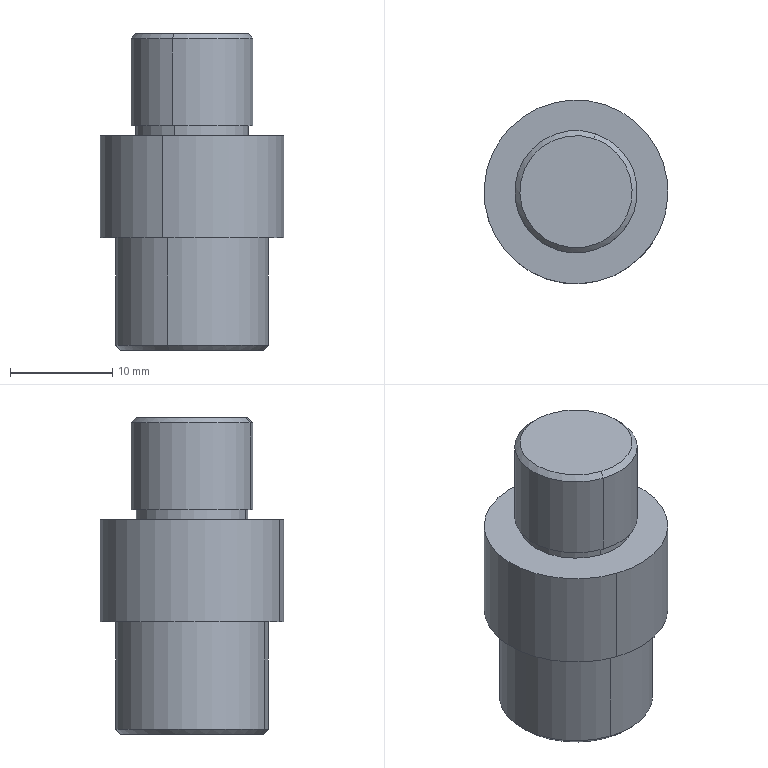Component | SolidWorks | 01-02WheelAxis-2 | 1 solid | 21 faces | box 18 x 18 x 31 mm | volume 5093 mm3 | cylinder 10 | cone 6 | plane 5 | commonest cylinder face diameters 6 x2 12 x2 11 x2 18 x2 15 x2 | material 45
build123d program:
from build123d import *

# Parameters (mm, degrees)
CHAMFER1_SIZE         = 0.5
M6_TAPPED_HOLE1_D     = 6
M6_TAPPED_HOLE1_DEPTH = 17
M6_TAPPED_HOLE1_TIP   = 1.803


with BuildPart() as part:
    # Sketch1 → Revolve1 (revolve)
    with BuildSketch(Plane.XY, mode=Mode.PRIVATE) as revolve1_sk:
        Polygon((0, 6), (0, 0), (31, 0), (31, 7.5), (20, 7.5), (20, 9), (10, 9), (10, 6), (10, 5.5), (9, 5.5), (9, 6), align=None)
    revolve(revolve1_sk.sketch.rotate(Axis((31, 0, 0), (-1, 0, 0)), 90), axis=Axis((31, 0, 0), (-1, 0, 0)))

    # Chamfer1
    chamfer1_edges = [part.edges().sort_by_distance(p)[0] for p in [
        (31, 0, 7.5),
        (0, 0, 6),
    ]]
    chamfer(chamfer1_edges, length=CHAMFER1_SIZE)

    # M6 Tapped Hole1
    with Locations(Plane(origin=(31, 0, 0), x_dir=(0, 0, -1), z_dir=(1, 0, 0))):
        with Locations((0, 0)):
            Hole(M6_TAPPED_HOLE1_D / 2, depth=M6_TAPPED_HOLE1_DEPTH)
            with Locations((0, 0, -(M6_TAPPED_HOLE1_DEPTH + M6_TAPPED_HOLE1_TIP / 2))):  # 118° drill point
                Cone(0, M6_TAPPED_HOLE1_D / 2, M6_TAPPED_HOLE1_TIP, mode=Mode.SUBTRACT)


solid = part.part

# Placed as in the assembly
solid = solid.moved(Location((300, -53.25, -443), (0, 90, 0)))
STEP:
#1=COLOUR_RGB('',0.7922,0.8196,0.9333);
#2=FILL_AREA_STYLE_COLOUR('',#1);
#3=FILL_AREA_STYLE('',(#2));
#4=SURFACE_STYLE_FILL_AREA(#3);
#5=SURFACE_SIDE_STYLE('',(#4));
#6=SURFACE_STYLE_USAGE(.BOTH.,#5);
#7=PRESENTATION_STYLE_ASSIGNMENT((#6));
#8=CARTESIAN_POINT('',(11.773,-2.208,-17.992));
#9=VERTEX_POINT('',#8);
#10=CARTESIAN_POINT('',(11.849,-1.985,-17.992));
#11=VERTEX_POINT('',#10);
#12=CARTESIAN_POINT('',(11.811,-2.096,-17.992));
#13=DIRECTION('',(0.,-0.,-1.));
#14=DIRECTION('',(0.3195,0.9476,0.));
#15=AXIS2_PLACEMENT_3D('',#12,#13,#14);
#16=CIRCLE('',#15,0.1181);
#17=EDGE_CURVE('',#9,#11,#16,.T.);
#18=ORIENTED_EDGE('',*,*,#17,.F.);
#19=CARTESIAN_POINT('',(11.773,-2.208,-18.661));
#20=VERTEX_POINT('',#19);
#21=CARTESIAN_POINT('',(11.773,-2.208,-18.661));
#22=DIRECTION('',(0.,-0.,-1.));
#23=VECTOR('',#22,39.37);
#24=LINE('',#21,#23);
#25=EDGE_CURVE('',#9,#20,#24,.T.);
#26=ORIENTED_EDGE('',*,*,#25,.T.);
#27=CARTESIAN_POINT('',(11.849,-1.985,-18.661));
#28=VERTEX_POINT('',#27);
#29=CARTESIAN_POINT('',(11.811,-2.096,-18.661));
#30=DIRECTION('',(0.,-0.,-1.));
#31=DIRECTION('',(0.3195,0.9476,0.));
#32=AXIS2_PLACEMENT_3D('',#29,#30,#31);
#33=CIRCLE('',#32,0.1181);
#34=EDGE_CURVE('',#20,#28,#33,.T.);
#35=ORIENTED_EDGE('',*,*,#34,.T.);
#36=CARTESIAN_POINT('',(11.849,-1.985,-18.661));
#37=DIRECTION('',(0.,-0.,-1.));
#38=VECTOR('',#37,39.37);
#39=LINE('',#36,#38);
#40=EDGE_CURVE('',#11,#28,#39,.T.);
#41=ORIENTED_EDGE('',*,*,#40,.F.);
#42=EDGE_LOOP('',(#18,#26,#35,#41));
#43=FACE_OUTER_BOUND('',#42,.T.);
#44=CARTESIAN_POINT('',(11.811,-2.096,-18.661));
#45=DIRECTION('',(0.,-0.,-1.));
#46=DIRECTION('',(0.3195,0.9476,0.));
#47=AXIS2_PLACEMENT_3D('',#44,#45,#46);
#48=CYLINDRICAL_SURFACE('',#47,0.1181);
#49=ADVANCED_FACE('',(#43),#48,.F.);
#50=CARTESIAN_POINT('',(11.811,-2.096,-17.921));
#51=VERTEX_POINT('',#50);
#52=CARTESIAN_POINT('',(11.849,-1.985,-17.992));
#53=DIRECTION('',(0.2739,0.8122,-0.515));
#54=VECTOR('',#53,39.37);
#55=LINE('',#52,#54);
#56=EDGE_CURVE('',#51,#11,#55,.T.);
#57=ORIENTED_EDGE('',*,*,#56,.F.);
#58=CARTESIAN_POINT('',(11.773,-2.208,-17.992));
#59=DIRECTION('',(-0.2739,-0.8122,-0.515));
#60=VECTOR('',#59,39.37);
#61=LINE('',#58,#60);
#62=EDGE_CURVE('',#51,#9,#61,.T.);
#63=ORIENTED_EDGE('',*,*,#62,.T.);
#64=ORIENTED_EDGE('',*,*,#17,.T.);
#65=EDGE_LOOP('',(#57,#63,#64));
#66=FACE_OUTER_BOUND('',#65,.T.);
#67=CARTESIAN_POINT('',(11.811,-2.096,-17.992));
#68=DIRECTION('',(0.,-0.,-1.));
#69=DIRECTION('',(0.3195,0.9476,0.));
#70=AXIS2_PLACEMENT_3D('',#67,#68,#69);
#71=CONICAL_SURFACE('',#70,0.1181,1.03);
#72=ADVANCED_FACE('',(#66),#71,.F.);
#73=CARTESIAN_POINT('',(11.899,-1.835,-18.661));
#74=VERTEX_POINT('',#73);
#75=CARTESIAN_POINT('',(11.723,-2.358,-18.661));
#76=VERTEX_POINT('',#75);
#77=CARTESIAN_POINT('',(11.811,-2.096,-18.661));
#78=DIRECTION('',(0.,-0.,-1.));
#79=DIRECTION('',(-0.3195,-0.9476,0.));
#80=AXIS2_PLACEMENT_3D('',#77,#78,#79);
#81=CIRCLE('',#80,0.2756);
#82=EDGE_CURVE('',#74,#76,#81,.T.);
#83=ORIENTED_EDGE('',*,*,#82,.F.);
#84=CARTESIAN_POINT('',(11.905,-1.817,-18.642));
#85=VERTEX_POINT('',#84);
#86=CARTESIAN_POINT('',(11.899,-1.835,-18.661));
#87=DIRECTION('',(0.2259,0.67,0.7071));
#88=VECTOR('',#87,39.37);
#89=LINE('',#86,#88);
#90=EDGE_CURVE('',#74,#85,#89,.T.);
#91=ORIENTED_EDGE('',*,*,#90,.T.);
#92=CARTESIAN_POINT('',(11.717,-2.376,-18.642));
#93=VERTEX_POINT('',#92);
#94=CARTESIAN_POINT('',(11.811,-2.096,-18.642));
#95=DIRECTION('',(-0.,0.,1.));
#96=DIRECTION('',(-0.3195,-0.9476,0.));
#97=AXIS2_PLACEMENT_3D('',#94,#95,#96);
#98=CIRCLE('',#97,0.2953);
#99=EDGE_CURVE('',#93,#85,#98,.T.);
#100=ORIENTED_EDGE('',*,*,#99,.F.);
#101=CARTESIAN_POINT('',(11.723,-2.358,-18.661));
#102=DIRECTION('',(-0.2259,-0.67,0.7071));
#103=VECTOR('',#102,39.37);
#104=LINE('',#101,#103);
#105=EDGE_CURVE('',#76,#93,#104,.T.);
#106=ORIENTED_EDGE('',*,*,#105,.F.);
#107=EDGE_LOOP('',(#83,#91,#100,#106));
#108=FACE_OUTER_BOUND('',#107,.T.);
#109=CARTESIAN_POINT('',(11.811,-2.096,-18.661));
#110=DIRECTION('',(-0.,0.,1.));
#111=DIRECTION('',(-0.3195,-0.9476,0.));
#112=AXIS2_PLACEMENT_3D('',#109,#110,#111);
#113=CONICAL_SURFACE('',#112,0.2756,0.7854);
#114=ADVANCED_FACE('',(#108),#113,.T.);
#115=CARTESIAN_POINT('',(11.742,-2.302,-17.441));
#116=VERTEX_POINT('',#115);
#117=CARTESIAN_POINT('',(11.88,-1.891,-17.441));
#118=VERTEX_POINT('',#117);
#119=CARTESIAN_POINT('',(11.811,-2.096,-17.441));
#120=DIRECTION('',(-0.,0.,1.));
#121=DIRECTION('',(0.3195,0.9476,0.));
#122=AXIS2_PLACEMENT_3D('',#119,#120,#121);
#123=CIRCLE('',#122,0.2165);
#124=EDGE_CURVE('',#116,#118,#123,.T.);
#125=ORIENTED_EDGE('',*,*,#124,.F.);
#126=CARTESIAN_POINT('',(11.736,-2.32,-17.461));
#127=VERTEX_POINT('',#126);
#128=CARTESIAN_POINT('',(11.736,-2.32,-17.461));
#129=DIRECTION('',(-0.2259,-0.67,-0.7071));
#130=VECTOR('',#129,39.37);
#131=LINE('',#128,#130);
#132=EDGE_CURVE('',#116,#127,#131,.T.);
#133=ORIENTED_EDGE('',*,*,#132,.T.);
#134=CARTESIAN_POINT('',(11.886,-1.873,-17.461));
#135=VERTEX_POINT('',#134);
#136=CARTESIAN_POINT('',(11.811,-2.096,-17.461));
#137=DIRECTION('',(0.,-0.,-1.));
#138=DIRECTION('',(0.3195,0.9476,0.));
#139=AXIS2_PLACEMENT_3D('',#136,#137,#138);
#140=CIRCLE('',#139,0.2362);
#141=EDGE_CURVE('',#135,#127,#140,.T.);
#142=ORIENTED_EDGE('',*,*,#141,.F.);
#143=CARTESIAN_POINT('',(11.886,-1.873,-17.461));
#144=DIRECTION('',(0.2259,0.67,-0.7071));
#145=VECTOR('',#144,39.37);
#146=LINE('',#143,#145);
#147=EDGE_CURVE('',#118,#135,#146,.T.);
#148=ORIENTED_EDGE('',*,*,#147,.F.);
#149=EDGE_LOOP('',(#125,#133,#142,#148));
#150=FACE_OUTER_BOUND('',#149,.T.);
#151=CARTESIAN_POINT('',(11.811,-2.096,-17.461));
#152=DIRECTION('',(0.,-0.,-1.));
#153=DIRECTION('',(0.3195,0.9476,0.));
#154=AXIS2_PLACEMENT_3D('',#151,#152,#153);
#155=CONICAL_SURFACE('',#154,0.2362,0.7854);
#156=ADVANCED_FACE('',(#150),#155,.T.);
#157=ORIENTED_EDGE('',*,*,#141,.T.);
#158=CARTESIAN_POINT('',(11.736,-2.32,-17.795));
#159=VERTEX_POINT('',#158);
#160=CARTESIAN_POINT('',(11.736,-2.32,-18.661));
#161=DIRECTION('',(0.,-0.,-1.));
#162=VECTOR('',#161,39.37);
#163=LINE('',#160,#162);
#164=EDGE_CURVE('',#127,#159,#163,.T.);
#165=ORIENTED_EDGE('',*,*,#164,.T.);
#166=CARTESIAN_POINT('',(11.886,-1.873,-17.795));
#167=VERTEX_POINT('',#166);
#168=CARTESIAN_POINT('',(11.811,-2.096,-17.795));
#169=DIRECTION('',(0.,-0.,-1.));
#170=DIRECTION('',(0.3195,0.9476,0.));
#171=AXIS2_PLACEMENT_3D('',#168,#169,#170);
#172=CIRCLE('',#171,0.2362);
#173=EDGE_CURVE('',#167,#159,#172,.T.);
#174=ORIENTED_EDGE('',*,*,#173,.F.);
#175=CARTESIAN_POINT('',(11.886,-1.873,-18.661));
#176=DIRECTION('',(0.,-0.,-1.));
#177=VECTOR('',#176,39.37);
#178=LINE('',#175,#177);
#179=EDGE_CURVE('',#135,#167,#178,.T.);
#180=ORIENTED_EDGE('',*,*,#179,.F.);
#181=EDGE_LOOP('',(#157,#165,#174,#180));
#182=FACE_OUTER_BOUND('',#181,.T.);
#183=CARTESIAN_POINT('',(11.811,-2.096,-18.661));
#184=DIRECTION('',(0.,-0.,-1.));
#185=DIRECTION('',(0.3195,0.9476,0.));
#186=AXIS2_PLACEMENT_3D('',#183,#184,#185);
#187=CYLINDRICAL_SURFACE('',#186,0.2362);
#188=ADVANCED_FACE('',(#182),#187,.T.);
#189=CARTESIAN_POINT('',(11.88,-1.891,-17.795));
#190=VERTEX_POINT('',#189);
#191=CARTESIAN_POINT('',(11.742,-2.302,-17.795));
#192=VERTEX_POINT('',#191);
#193=CARTESIAN_POINT('',(11.811,-2.096,-17.795));
#194=DIRECTION('',(0.,-0.,-1.));
#195=DIRECTION('',(0.3195,0.9476,0.));
#196=AXIS2_PLACEMENT_3D('',#193,#194,#195);
#197=CIRCLE('',#196,0.2165);
#198=EDGE_CURVE('',#190,#192,#197,.T.);
#199=ORIENTED_EDGE('',*,*,#198,.T.);
#200=CARTESIAN_POINT('',(11.742,-2.302,-17.835));
#201=VERTEX_POINT('',#200);
#202=CARTESIAN_POINT('',(11.742,-2.302,-18.661));
#203=DIRECTION('',(0.,-0.,-1.));
#204=VECTOR('',#203,39.37);
#205=LINE('',#202,#204);
#206=EDGE_CURVE('',#192,#201,#205,.T.);
#207=ORIENTED_EDGE('',*,*,#206,.T.);
#208=CARTESIAN_POINT('',(11.88,-1.891,-17.835));
#209=VERTEX_POINT('',#208);
#210=CARTESIAN_POINT('',(11.811,-2.096,-17.835));
#211=DIRECTION('',(0.,-0.,-1.));
#212=DIRECTION('',(0.3195,0.9476,0.));
#213=AXIS2_PLACEMENT_3D('',#210,#211,#212);
#214=CIRCLE('',#213,0.2165);
#215=EDGE_CURVE('',#209,#201,#214,.T.);
#216=ORIENTED_EDGE('',*,*,#215,.F.);
#217=CARTESIAN_POINT('',(11.88,-1.891,-18.661));
#218=DIRECTION('',(0.,-0.,-1.));
#219=VECTOR('',#218,39.37);
#220=LINE('',#217,#219);
#221=EDGE_CURVE('',#190,#209,#220,.T.);
#222=ORIENTED_EDGE('',*,*,#221,.F.);
#223=EDGE_LOOP('',(#199,#207,#216,#222));
#224=FACE_OUTER_BOUND('',#223,.T.);
#225=CARTESIAN_POINT('',(11.811,-2.096,-18.661));
#226=DIRECTION('',(0.,-0.,-1.));
#227=DIRECTION('',(0.3195,0.9476,0.));
#228=AXIS2_PLACEMENT_3D('',#225,#226,#227);
#229=CYLINDRICAL_SURFACE('',#228,0.2165);
#230=ADVANCED_FACE('',(#224),#229,.T.);
#231=CARTESIAN_POINT('',(11.924,-1.761,-17.835));
#232=VERTEX_POINT('',#231);
#233=CARTESIAN_POINT('',(11.698,-2.432,-17.835));
#234=VERTEX_POINT('',#233);
#235=CARTESIAN_POINT('',(11.811,-2.096,-17.835));
#236=DIRECTION('',(0.,-0.,-1.));
#237=DIRECTION('',(0.3195,0.9476,0.));
#238=AXIS2_PLACEMENT_3D('',#235,#236,#237);
#239=CIRCLE('',#238,0.3543);
#240=EDGE_CURVE('',#232,#234,#239,.T.);
#241=ORIENTED_EDGE('',*,*,#240,.T.);
#242=CARTESIAN_POINT('',(11.698,-2.432,-18.228));
#243=VERTEX_POINT('',#242);
#244=CARTESIAN_POINT('',(11.698,-2.432,-18.661));
#245=DIRECTION('',(0.,-0.,-1.));
#246=VECTOR('',#245,39.37);
#247=LINE('',#244,#246);
#248=EDGE_CURVE('',#234,#243,#247,.T.);
#249=ORIENTED_EDGE('',*,*,#248,.T.);
#250=CARTESIAN_POINT('',(11.924,-1.761,-18.228));
#251=VERTEX_POINT('',#250);
#252=CARTESIAN_POINT('',(11.811,-2.096,-18.228));
#253=DIRECTION('',(0.,-0.,-1.));
#254=DIRECTION('',(0.3195,0.9476,0.));
#255=AXIS2_PLACEMENT_3D('',#252,#253,#254);
#256=CIRCLE('',#255,0.3543);
#257=EDGE_CURVE('',#251,#243,#256,.T.);
#258=ORIENTED_EDGE('',*,*,#257,.F.);
#259=CARTESIAN_POINT('',(11.924,-1.761,-18.661));
#260=DIRECTION('',(0.,-0.,-1.));
#261=VECTOR('',#260,39.37);
#262=LINE('',#259,#261);
#263=EDGE_CURVE('',#232,#251,#262,.T.);
#264=ORIENTED_EDGE('',*,*,#263,.F.);
#265=EDGE_LOOP('',(#241,#249,#258,#264));
#266=FACE_OUTER_BOUND('',#265,.T.);
#267=CARTESIAN_POINT('',(11.811,-2.096,-18.661));
#268=DIRECTION('',(0.,-0.,-1.));
#269=DIRECTION('',(0.3195,0.9476,0.));
#270=AXIS2_PLACEMENT_3D('',#267,#268,#269);
#271=CYLINDRICAL_SURFACE('',#270,0.3543);
#272=ADVANCED_FACE('',(#266),#271,.T.);
#273=CARTESIAN_POINT('',(11.905,-1.817,-18.228));
#274=VERTEX_POINT('',#273);
#275=CARTESIAN_POINT('',(11.717,-2.376,-18.228));
#276=VERTEX_POINT('',#275);
#277=CARTESIAN_POINT('',(11.811,-2.096,-18.228));
#278=DIRECTION('',(0.,-0.,-1.));
#279=DIRECTION('',(0.3195,0.9476,0.));
#280=AXIS2_PLACEMENT_3D('',#277,#278,#279);
#281=CIRCLE('',#280,0.2953);
#282=EDGE_CURVE('',#274,#276,#281,.T.);
#283=ORIENTED_EDGE('',*,*,#282,.T.);
#284=CARTESIAN_POINT('',(11.717,-2.376,-18.661));
#285=DIRECTION('',(0.,-0.,-1.));
#286=VECTOR('',#285,39.37);
#287=LINE('',#284,#286);
#288=EDGE_CURVE('',#276,#93,#287,.T.);
#289=ORIENTED_EDGE('',*,*,#288,.T.);
#290=ORIENTED_EDGE('',*,*,#99,.T.);
#291=CARTESIAN_POINT('',(11.905,-1.817,-18.661));
#292=DIRECTION('',(0.,-0.,-1.));
#293=VECTOR('',#292,39.37);
#294=LINE('',#291,#293);
#295=EDGE_CURVE('',#274,#85,#294,.T.);
#296=ORIENTED_EDGE('',*,*,#295,.F.);
#297=EDGE_LOOP('',(#283,#289,#290,#296));
#298=FACE_OUTER_BOUND('',#297,.T.);
#299=CARTESIAN_POINT('',(11.811,-2.096,-18.661));
#300=DIRECTION('',(0.,-0.,-1.));
#301=DIRECTION('',(0.3195,0.9476,0.));
#302=AXIS2_PLACEMENT_3D('',#299,#300,#301);
#303=CYLINDRICAL_SURFACE('',#302,0.2953);
#304=ADVANCED_FACE('',(#298),#303,.T.);
#305=CARTESIAN_POINT('',(11.811,-2.096,-18.661));
#306=DIRECTION('',(0.,-0.,-1.));
#307=DIRECTION('',(0.3195,0.9476,0.));
#308=AXIS2_PLACEMENT_3D('',#305,#306,#307);
#309=CIRCLE('',#308,0.1181);
#310=EDGE_CURVE('',#28,#20,#309,.T.);
#311=ORIENTED_EDGE('',*,*,#310,.F.);
#312=ORIENTED_EDGE('',*,*,#34,.F.);
#313=EDGE_LOOP('',(#311,#312));
#314=FACE_BOUND('',#313,.T.);
#315=CARTESIAN_POINT('',(11.811,-2.096,-18.661));
#316=DIRECTION('',(0.,-0.,-1.));
#317=DIRECTION('',(-0.3195,-0.9476,0.));
#318=AXIS2_PLACEMENT_3D('',#315,#316,#317);
#319=CIRCLE('',#318,0.2756);
#320=EDGE_CURVE('',#76,#74,#319,.T.);
#321=ORIENTED_EDGE('',*,*,#320,.T.);
#322=ORIENTED_EDGE('',*,*,#82,.T.);
#323=EDGE_LOOP('',(#321,#322));
#324=FACE_OUTER_BOUND('',#323,.T.);
#325=CARTESIAN_POINT('',(11.811,-2.096,-18.661));
#326=DIRECTION('',(-0.,0.,1.));
#327=DIRECTION('',(-0.3195,-0.9476,-0.));
#328=AXIS2_PLACEMENT_3D('',#325,#326,#327);
#329=PLANE('',#328);
#330=ADVANCED_FACE('',(#314,#324),#329,.F.);
#331=ORIENTED_EDGE('',*,*,#288,.F.);
#332=CARTESIAN_POINT('',(11.811,-2.096,-18.228));
#333=DIRECTION('',(0.,-0.,-1.));
#334=DIRECTION('',(0.3195,0.9476,0.));
#335=AXIS2_PLACEMENT_3D('',#332,#333,#334);
#336=CIRCLE('',#335,0.2953);
#337=EDGE_CURVE('',#276,#274,#336,.T.);
#338=ORIENTED_EDGE('',*,*,#337,.T.);
#339=ORIENTED_EDGE('',*,*,#295,.T.);
#340=CARTESIAN_POINT('',(11.811,-2.096,-18.642));
#341=DIRECTION('',(-0.,0.,1.));
#342=DIRECTION('',(-0.3195,-0.9476,0.));
#343=AXIS2_PLACEMENT_3D('',#340,#341,#342);
#344=CIRCLE('',#343,0.2953);
#345=EDGE_CURVE('',#85,#93,#344,.T.);
#346=ORIENTED_EDGE('',*,*,#345,.T.);
#347=EDGE_LOOP('',(#331,#338,#339,#346));
#348=FACE_OUTER_BOUND('',#347,.T.);
#349=CARTESIAN_POINT('',(11.811,-2.096,-18.661));
#350=DIRECTION('',(0.,-0.,-1.));
#351=DIRECTION('',(0.3195,0.9476,0.));
#352=AXIS2_PLACEMENT_3D('',#349,#350,#351);
#353=CYLINDRICAL_SURFACE('',#352,0.2953);
#354=ADVANCED_FACE('',(#348),#353,.T.);
#355=ORIENTED_EDGE('',*,*,#282,.F.);
#356=ORIENTED_EDGE('',*,*,#337,.F.);
#357=EDGE_LOOP('',(#355,#356));
#358=FACE_BOUND('',#357,.T.);
#359=ORIENTED_EDGE('',*,*,#257,.T.);
#360=CARTESIAN_POINT('',(11.811,-2.096,-18.228));
#361=DIRECTION('',(0.,-0.,-1.));
#362=DIRECTION('',(0.3195,0.9476,0.));
#363=AXIS2_PLACEMENT_3D('',#360,#361,#362);
#364=CIRCLE('',#363,0.3543);
#365=EDGE_CURVE('',#243,#251,#364,.T.);
#366=ORIENTED_EDGE('',*,*,#365,.T.);
#367=EDGE_LOOP('',(#359,#366));
#368=FACE_OUTER_BOUND('',#367,.T.);
#369=CARTESIAN_POINT('',(11.811,-2.096,-18.228));
#370=DIRECTION('',(-0.,0.,1.));
#371=DIRECTION('',(-0.3195,-0.9476,-0.));
#372=AXIS2_PLACEMENT_3D('',#369,#370,#371);
#373=PLANE('',#372);
#374=ADVANCED_FACE('',(#358,#368),#373,.F.);
#375=ORIENTED_EDGE('',*,*,#248,.F.);
#376=CARTESIAN_POINT('',(11.811,-2.096,-17.835));
#377=DIRECTION('',(0.,-0.,-1.));
#378=DIRECTION('',(0.3195,0.9476,0.));
#379=AXIS2_PLACEMENT_3D('',#376,#377,#378);
#380=CIRCLE('',#379,0.3543);
#381=EDGE_CURVE('',#234,#232,#380,.T.);
#382=ORIENTED_EDGE('',*,*,#381,.T.);
#383=ORIENTED_EDGE('',*,*,#263,.T.);
#384=ORIENTED_EDGE('',*,*,#365,.F.);
#385=EDGE_LOOP('',(#375,#382,#383,#384));
#386=FACE_OUTER_BOUND('',#385,.T.);
#387=CARTESIAN_POINT('',(11.811,-2.096,-18.661));
#388=DIRECTION('',(0.,-0.,-1.));
#389=DIRECTION('',(0.3195,0.9476,0.));
#390=AXIS2_PLACEMENT_3D('',#387,#388,#389);
#391=CYLINDRICAL_SURFACE('',#390,0.3543);
#392=ADVANCED_FACE('',(#386),#391,.T.);
#393=ORIENTED_EDGE('',*,*,#240,.F.);
#394=ORIENTED_EDGE('',*,*,#381,.F.);
#395=EDGE_LOOP('',(#393,#394));
#396=FACE_OUTER_BOUND('',#395,.T.);
#397=ORIENTED_EDGE('',*,*,#215,.T.);
#398=CARTESIAN_POINT('',(11.811,-2.096,-17.835));
#399=DIRECTION('',(0.,-0.,-1.));
#400=DIRECTION('',(0.3195,0.9476,0.));
#401=AXIS2_PLACEMENT_3D('',#398,#399,#400);
#402=CIRCLE('',#401,0.2165);
#403=EDGE_CURVE('',#201,#209,#402,.T.);
#404=ORIENTED_EDGE('',*,*,#403,.T.);
#405=EDGE_LOOP('',(#397,#404));
#406=FACE_BOUND('',#405,.T.);
#407=CARTESIAN_POINT('',(11.811,-2.096,-17.835));
#408=DIRECTION('',(0.,-0.,-1.));
#409=DIRECTION('',(0.3195,0.9476,0.));
#410=AXIS2_PLACEMENT_3D('',#407,#408,#409);
#411=PLANE('',#410);
#412=ADVANCED_FACE('',(#396,#406),#411,.F.);
#413=ORIENTED_EDGE('',*,*,#206,.F.);
#414=CARTESIAN_POINT('',(11.811,-2.096,-17.795));
#415=DIRECTION('',(0.,-0.,-1.));
#416=DIRECTION('',(0.3195,0.9476,0.));
#417=AXIS2_PLACEMENT_3D('',#414,#415,#416);
#418=CIRCLE('',#417,0.2165);
#419=EDGE_CURVE('',#192,#190,#418,.T.);
#420=ORIENTED_EDGE('',*,*,#419,.T.);
#421=ORIENTED_EDGE('',*,*,#221,.T.);
#422=ORIENTED_EDGE('',*,*,#403,.F.);
#423=EDGE_LOOP('',(#413,#420,#421,#422));
#424=FACE_OUTER_BOUND('',#423,.T.);
#425=CARTESIAN_POINT('',(11.811,-2.096,-18.661));
#426=DIRECTION('',(0.,-0.,-1.));
#427=DIRECTION('',(0.3195,0.9476,0.));
#428=AXIS2_PLACEMENT_3D('',#425,#426,#427);
#429=CYLINDRICAL_SURFACE('',#428,0.2165);
#430=ADVANCED_FACE('',(#424),#429,.T.);
#431=ORIENTED_EDGE('',*,*,#173,.T.);
#432=CARTESIAN_POINT('',(11.811,-2.096,-17.795));
#433=DIRECTION('',(0.,-0.,-1.));
#434=DIRECTION('',(0.3195,0.9476,0.));
#435=AXIS2_PLACEMENT_3D('',#432,#433,#434);
#436=CIRCLE('',#435,0.2362);
#437=EDGE_CURVE('',#159,#167,#436,.T.);
#438=ORIENTED_EDGE('',*,*,#437,.T.);
#439=EDGE_LOOP('',(#431,#438));
#440=FACE_OUTER_BOUND('',#439,.T.);
#441=ORIENTED_EDGE('',*,*,#198,.F.);
#442=ORIENTED_EDGE('',*,*,#419,.F.);
#443=EDGE_LOOP('',(#441,#442));
#444=FACE_BOUND('',#443,.T.);
#445=CARTESIAN_POINT('',(11.811,-2.096,-17.795));
#446=DIRECTION('',(0.,-0.,-1.));
#447=DIRECTION('',(0.3195,0.9476,0.));
#448=AXIS2_PLACEMENT_3D('',#445,#446,#447);
#449=PLANE('',#448);
#450=ADVANCED_FACE('',(#440,#444),#449,.T.);
#451=ORIENTED_EDGE('',*,*,#164,.F.);
#452=CARTESIAN_POINT('',(11.811,-2.096,-17.461));
#453=DIRECTION('',(0.,-0.,-1.));
#454=DIRECTION('',(0.3195,0.9476,0.));
#455=AXIS2_PLACEMENT_3D('',#452,#453,#454);
#456=CIRCLE('',#455,0.2362);
#457=EDGE_CURVE('',#127,#135,#456,.T.);
#458=ORIENTED_EDGE('',*,*,#457,.T.);
#459=ORIENTED_EDGE('',*,*,#179,.T.);
#460=ORIENTED_EDGE('',*,*,#437,.F.);
#461=EDGE_LOOP('',(#451,#458,#459,#460));
#462=FACE_OUTER_BOUND('',#461,.T.);
#463=CARTESIAN_POINT('',(11.811,-2.096,-18.661));
#464=DIRECTION('',(0.,-0.,-1.));
#465=DIRECTION('',(0.3195,0.9476,0.));
#466=AXIS2_PLACEMENT_3D('',#463,#464,#465);
#467=CYLINDRICAL_SURFACE('',#466,0.2362);
#468=ADVANCED_FACE('',(#462),#467,.T.);
#469=CARTESIAN_POINT('',(11.811,-2.096,-17.441));
#470=DIRECTION('',(-0.,0.,1.));
#471=DIRECTION('',(0.3195,0.9476,0.));
#472=AXIS2_PLACEMENT_3D('',#469,#470,#471);
#473=CIRCLE('',#472,0.2165);
#474=EDGE_CURVE('',#118,#116,#473,.T.);
#475=ORIENTED_EDGE('',*,*,#474,.T.);
#476=ORIENTED_EDGE('',*,*,#124,.T.);
#477=EDGE_LOOP('',(#475,#476));
#478=FACE_OUTER_BOUND('',#477,.T.);
#479=CARTESIAN_POINT('',(11.811,-2.096,-17.441));
#480=DIRECTION('',(0.,-0.,-1.));
#481=DIRECTION('',(0.3195,0.9476,0.));
#482=AXIS2_PLACEMENT_3D('',#479,#480,#481);
#483=PLANE('',#482);
#484=ADVANCED_FACE('',(#478),#483,.F.);
#485=ORIENTED_EDGE('',*,*,#132,.F.);
#486=ORIENTED_EDGE('',*,*,#474,.F.);
#487=ORIENTED_EDGE('',*,*,#147,.T.);
#488=ORIENTED_EDGE('',*,*,#457,.F.);
#489=EDGE_LOOP('',(#485,#486,#487,#488));
#490=FACE_OUTER_BOUND('',#489,.T.);
#491=CARTESIAN_POINT('',(11.811,-2.096,-17.461));
#492=DIRECTION('',(0.,-0.,-1.));
#493=DIRECTION('',(0.3195,0.9476,0.));
#494=AXIS2_PLACEMENT_3D('',#491,#492,#493);
#495=CONICAL_SURFACE('',#494,0.2362,0.7854);
#496=ADVANCED_FACE('',(#490),#495,.T.);
#497=ORIENTED_EDGE('',*,*,#90,.F.);
#498=ORIENTED_EDGE('',*,*,#320,.F.);
#499=ORIENTED_EDGE('',*,*,#105,.T.);
#500=ORIENTED_EDGE('',*,*,#345,.F.);
#501=EDGE_LOOP('',(#497,#498,#499,#500));
#502=FACE_OUTER_BOUND('',#501,.T.);
#503=CARTESIAN_POINT('',(11.811,-2.096,-18.661));
#504=DIRECTION('',(-0.,0.,1.));
#505=DIRECTION('',(-0.3195,-0.9476,0.));
#506=AXIS2_PLACEMENT_3D('',#503,#504,#505);
#507=CONICAL_SURFACE('',#506,0.2756,0.7854);
#508=ADVANCED_FACE('',(#502),#507,.T.);
#509=ORIENTED_EDGE('',*,*,#62,.F.);
#510=ORIENTED_EDGE('',*,*,#56,.T.);
#511=CARTESIAN_POINT('',(11.811,-2.096,-17.992));
#512=DIRECTION('',(0.,-0.,-1.));
#513=DIRECTION('',(0.3195,0.9476,0.));
#514=AXIS2_PLACEMENT_3D('',#511,#512,#513);
#515=CIRCLE('',#514,0.1181);
#516=EDGE_CURVE('',#11,#9,#515,.T.);
#517=ORIENTED_EDGE('',*,*,#516,.T.);
#518=EDGE_LOOP('',(#509,#510,#517));
#519=FACE_OUTER_BOUND('',#518,.T.);
#520=CARTESIAN_POINT('',(11.811,-2.096,-17.992));
#521=DIRECTION('',(0.,-0.,-1.));
#522=DIRECTION('',(0.3195,0.9476,0.));
#523=AXIS2_PLACEMENT_3D('',#520,#521,#522);
#524=CONICAL_SURFACE('',#523,0.1181,1.03);
#525=ADVANCED_FACE('',(#519),#524,.F.);
#526=ORIENTED_EDGE('',*,*,#25,.F.);
#527=ORIENTED_EDGE('',*,*,#516,.F.);
#528=ORIENTED_EDGE('',*,*,#40,.T.);
#529=ORIENTED_EDGE('',*,*,#310,.T.);
#530=EDGE_LOOP('',(#526,#527,#528,#529));
#531=FACE_OUTER_BOUND('',#530,.T.);
#532=CARTESIAN_POINT('',(11.811,-2.096,-18.661));
#533=DIRECTION('',(0.,-0.,-1.));
#534=DIRECTION('',(0.3195,0.9476,0.));
#535=AXIS2_PLACEMENT_3D('',#532,#533,#534);
#536=CYLINDRICAL_SURFACE('',#535,0.1181);
#537=ADVANCED_FACE('',(#531),#536,.F.);
#538=CLOSED_SHELL('',(#49,#72,#114,#156,#188,#230,#272,#304,#330,#354,#374,#392,#412,#430,#450,#468,#484,#496,#508,#525,#537));
#539=MANIFOLD_SOLID_BREP('',#538);
#540=STYLED_ITEM('',(#7),#539);
#541=(LENGTH_UNIT()NAMED_UNIT(*)SI_UNIT($,.METRE.));
#542=LENGTH_MEASURE_WITH_UNIT(LENGTH_MEASURE(0.0254),#541);
#543=DIMENSIONAL_EXPONENTS(1.,0.,0.,0.,0.,0.,0.);
#544=(CONVERSION_BASED_UNIT('',#542)LENGTH_UNIT()NAMED_UNIT(#543));
#545=UNCERTAINTY_MEASURE_WITH_UNIT(LENGTH_MEASURE(0.00001),#544,'','');
#546=(NAMED_UNIT(*)PLANE_ANGLE_UNIT()SI_UNIT($,.RADIAN.));
#547=(NAMED_UNIT(*)SI_UNIT($,.STERADIAN.)SOLID_ANGLE_UNIT());
#548=(GEOMETRIC_REPRESENTATION_CONTEXT(3)GLOBAL_UNCERTAINTY_ASSIGNED_CONTEXT((#545))GLOBAL_UNIT_ASSIGNED_CONTEXT((#544,#546,#547))REPRESENTATION_CONTEXT('',''));
#549=MECHANICAL_DESIGN_GEOMETRIC_PRESENTATION_REPRESENTATION('',(#540),#548);
#550=CARTESIAN_POINT('',(0.,0.,0.));
#551=DIRECTION('',(0.,0.,1.));
#552=DIRECTION('',(1.,0.,0.));
#553=AXIS2_PLACEMENT_3D('',#550,#551,#552);
#554=(LENGTH_UNIT()NAMED_UNIT(*)SI_UNIT($,.METRE.));
#555=LENGTH_MEASURE_WITH_UNIT(LENGTH_MEASURE(0.0254),#554);
#556=DIMENSIONAL_EXPONENTS(1.,0.,0.,0.,0.,0.,0.);
#557=(CONVERSION_BASED_UNIT('',#555)LENGTH_UNIT()NAMED_UNIT(#556));
#558=UNCERTAINTY_MEASURE_WITH_UNIT(LENGTH_MEASURE(0.00001),#557,'','');
#559=(NAMED_UNIT(*)PLANE_ANGLE_UNIT()SI_UNIT($,.RADIAN.));
#560=(NAMED_UNIT(*)SI_UNIT($,.STERADIAN.)SOLID_ANGLE_UNIT());
#561=(GEOMETRIC_REPRESENTATION_CONTEXT(3)GLOBAL_UNCERTAINTY_ASSIGNED_CONTEXT((#558))GLOBAL_UNIT_ASSIGNED_CONTEXT((#557,#559,#560))REPRESENTATION_CONTEXT('',''));
#562=ADVANCED_BREP_SHAPE_REPRESENTATION('',(#539,#553),#561);
#563=PRESENTATION_LAYER_ASSIGNMENT('','',(#540));